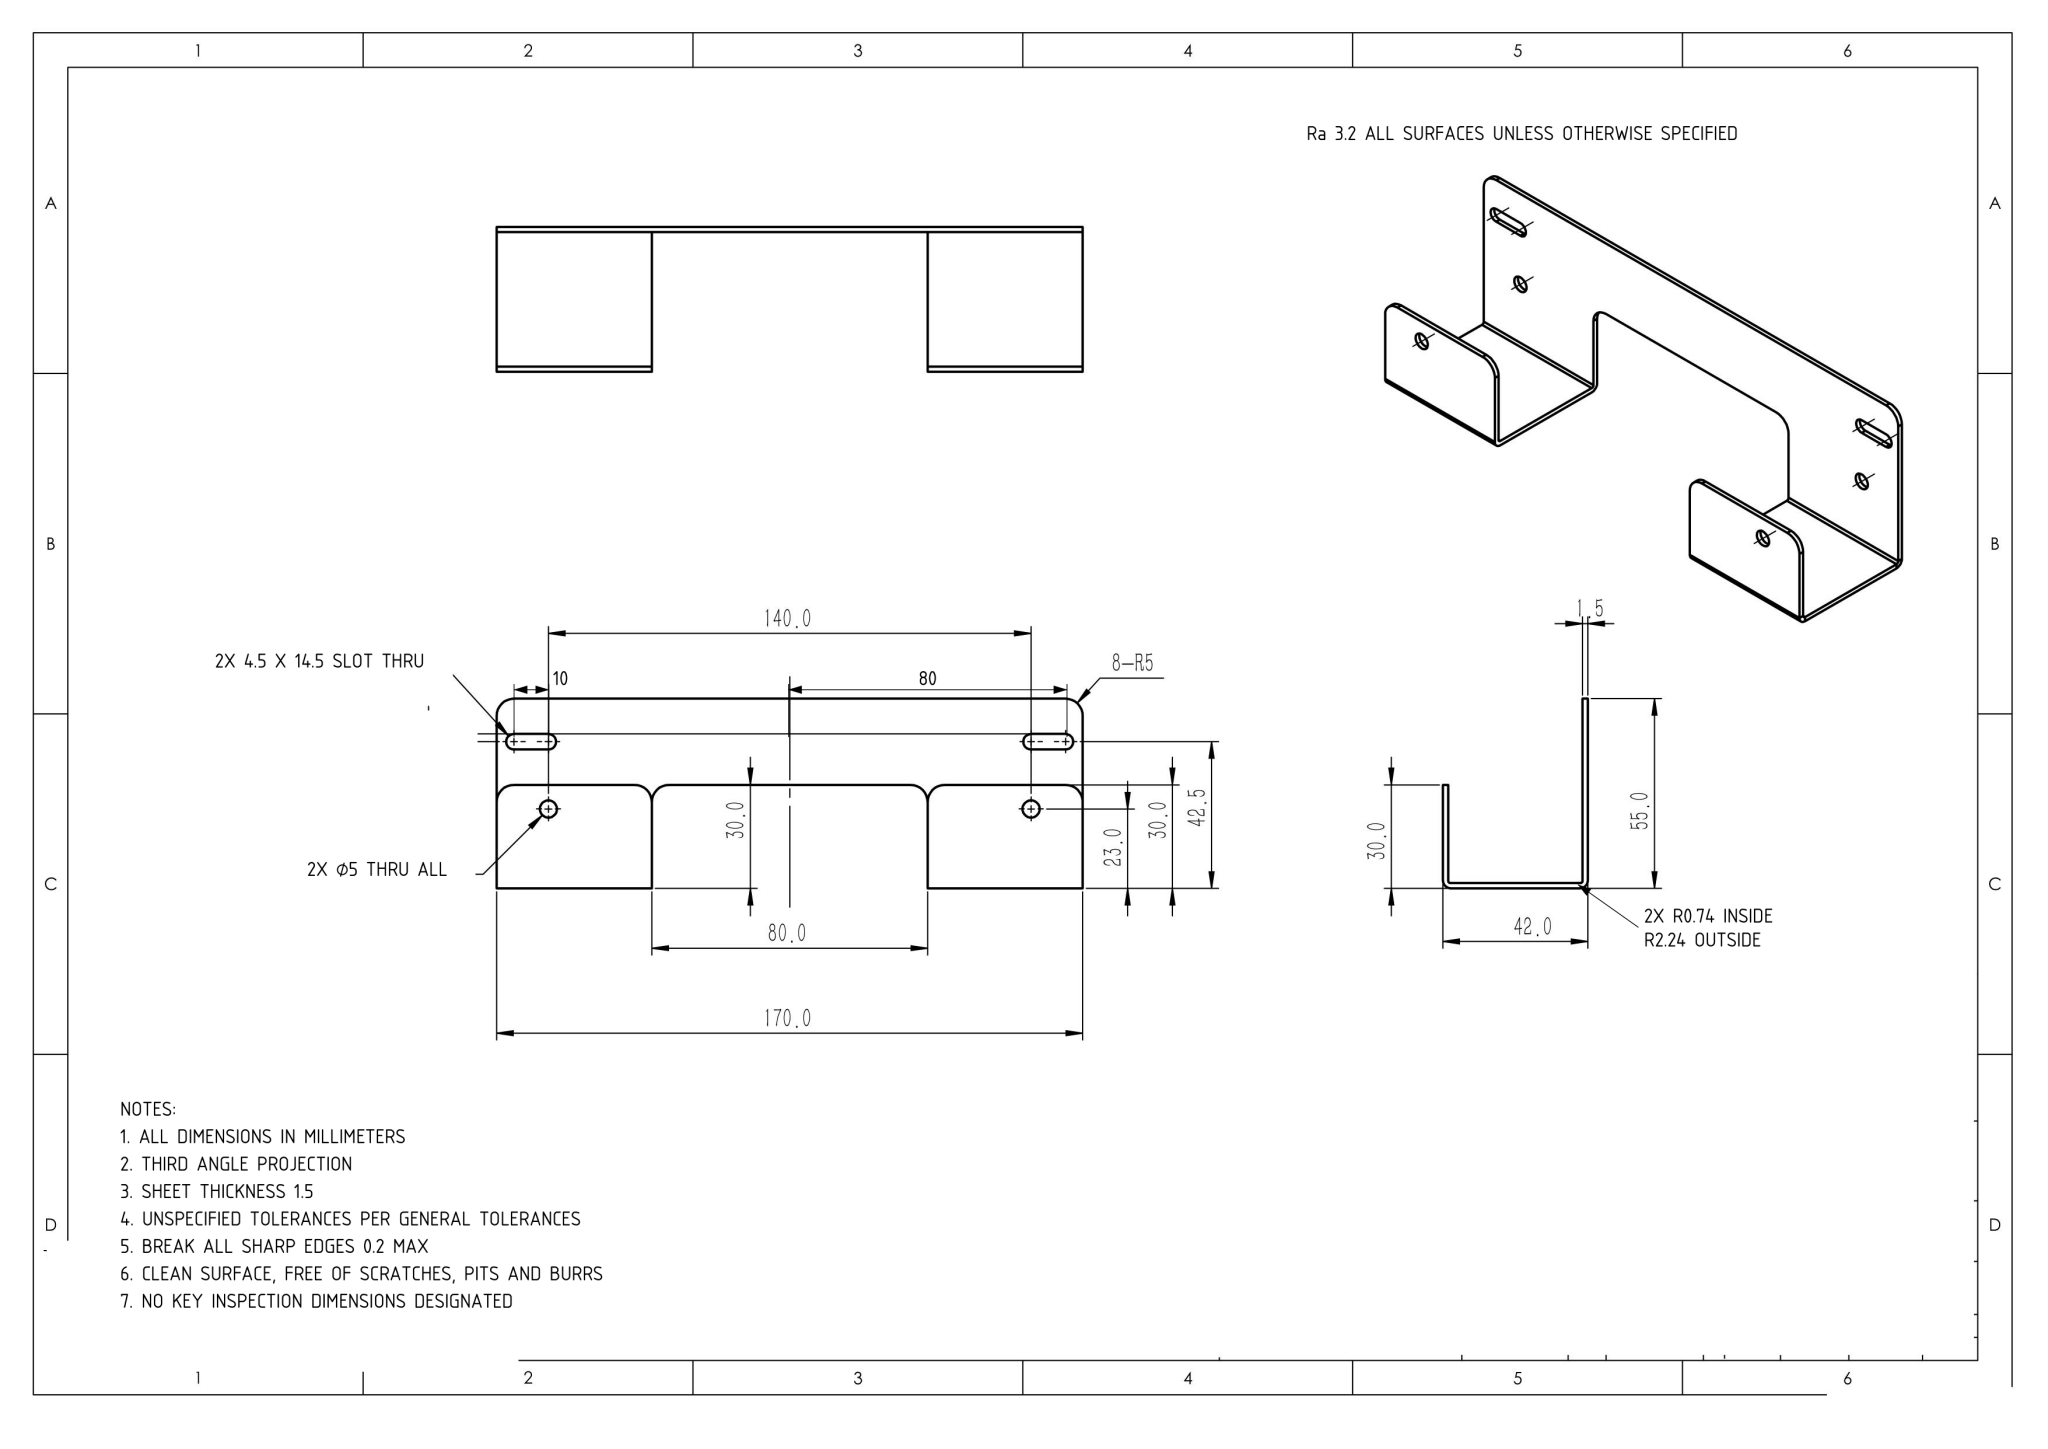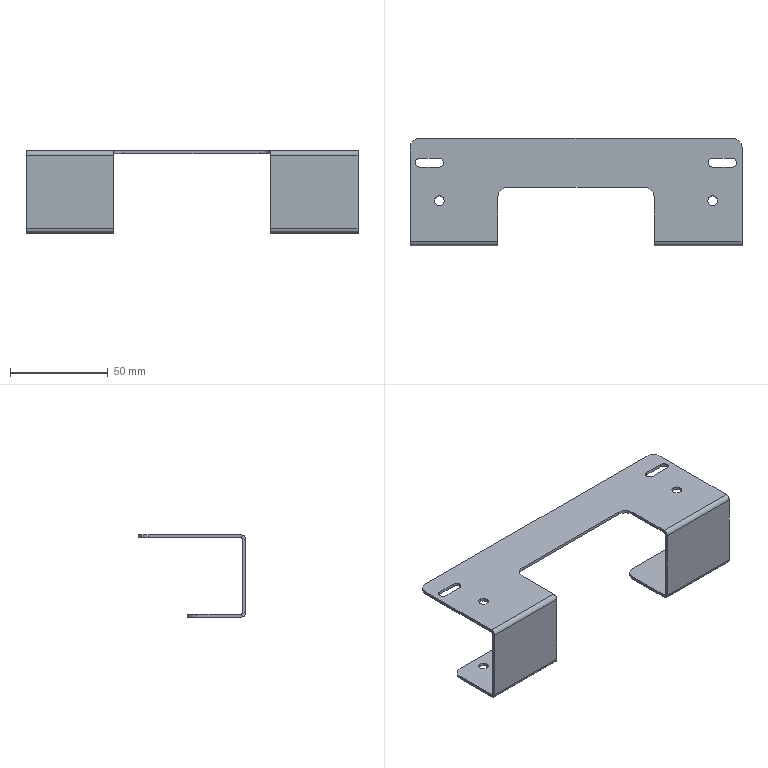Part | NX | mm | 1 solid | 60 faces | box 170 x 55 x 42 mm | volume 19235 mm3 | cylinder 30 | plane 30 | commonest cylinder face diameters 5 x8 10 x8 4.5 x6 4.473 x4 1.473 x4